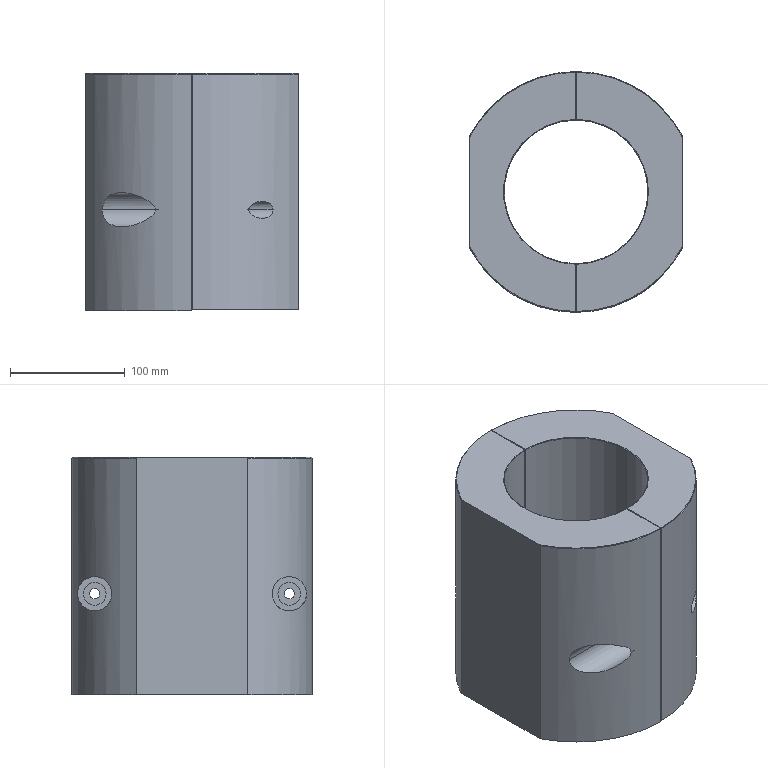Component | SolidWorks | ZN-A-010-1 | 2 solids | 123 faces | volume 3980488 mm3 | cylinder 68 | cone 33 | plane 22 | commonest cylinder face diameters 6.8 x14 12 x12 4.2 x8 30 x4 32 x4 8 x4 210 x4 9 x4